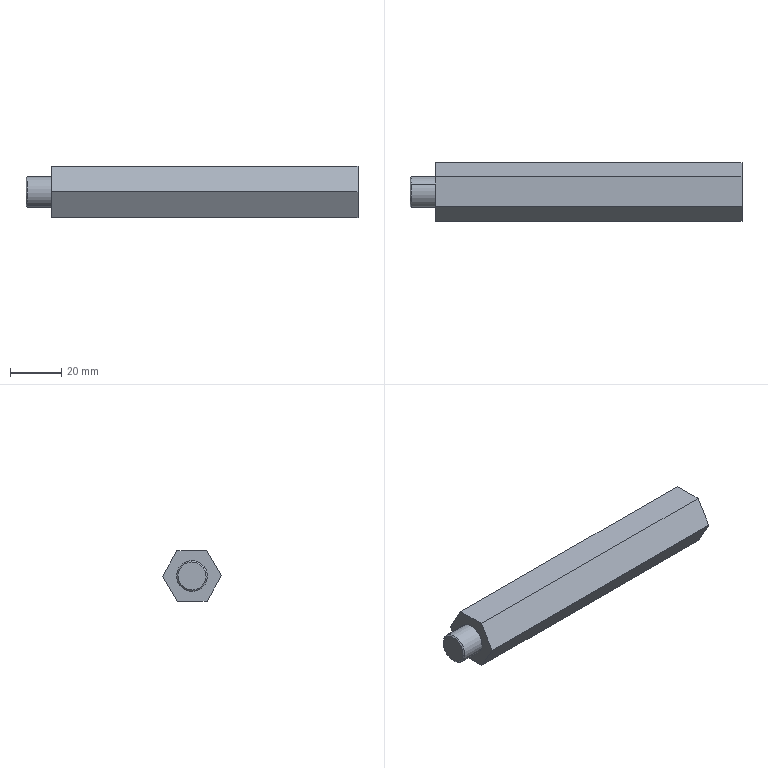Component | SolidWorks | LowerSideBeltXG-XG1-1_RollerMountingPlateABConnectingRodXG-XG1-1 | 1 solid | 17 faces | box 130 x 23.09 x 20.14 mm | volume 41863 mm3 | plane 9 | cone 4 | cylinder 4 | commonest cylinder face diameters 12 x2 6.8 x2
STEP:
#1=COLOUR_RGB('',0.7922,0.8196,0.9333);
#2=FILL_AREA_STYLE_COLOUR('',#1);
#3=FILL_AREA_STYLE('',(#2));
#4=SURFACE_STYLE_FILL_AREA(#3);
#5=SURFACE_SIDE_STYLE('',(#4));
#6=SURFACE_STYLE_USAGE(.BOTH.,#5);
#7=PRESENTATION_STYLE_ASSIGNMENT((#6));
#8=CARTESIAN_POINT('',(-12.843,21.445,3.515));
#9=VERTEX_POINT('',#8);
#10=CARTESIAN_POINT('',(-12.843,21.666,3.887));
#11=VERTEX_POINT('',#10);
#12=CARTESIAN_POINT('',(-12.843,21.555,3.701));
#13=DIRECTION('',(-1.,-0.,0.));
#14=DIRECTION('',(0.,-0.5106,-0.8598));
#15=AXIS2_PLACEMENT_3D('',#12,#13,#14);
#16=CIRCLE('',#15,0.2165);
#17=EDGE_CURVE('',#9,#11,#16,.T.);
#18=ORIENTED_EDGE('',*,*,#17,.F.);
#19=CARTESIAN_POINT('',(-12.824,21.434,3.498));
#20=VERTEX_POINT('',#19);
#21=CARTESIAN_POINT('',(-12.843,21.445,3.515));
#22=DIRECTION('',(0.7071,-0.3611,-0.608));
#23=VECTOR('',#22,39.37);
#24=LINE('',#21,#23);
#25=EDGE_CURVE('',#9,#20,#24,.T.);
#26=ORIENTED_EDGE('',*,*,#25,.T.);
#27=CARTESIAN_POINT('',(-12.824,21.676,3.904));
#28=VERTEX_POINT('',#27);
#29=CARTESIAN_POINT('',(-12.824,21.555,3.701));
#30=DIRECTION('',(1.,0.,-0.));
#31=DIRECTION('',(0.,-0.5106,-0.8598));
#32=AXIS2_PLACEMENT_3D('',#29,#30,#31);
#33=CIRCLE('',#32,0.2362);
#34=EDGE_CURVE('',#28,#20,#33,.T.);
#35=ORIENTED_EDGE('',*,*,#34,.F.);
#36=CARTESIAN_POINT('',(-12.843,21.666,3.887));
#37=DIRECTION('',(0.7071,0.3611,0.608));
#38=VECTOR('',#37,39.37);
#39=LINE('',#36,#38);
#40=EDGE_CURVE('',#11,#28,#39,.T.);
#41=ORIENTED_EDGE('',*,*,#40,.F.);
#42=EDGE_LOOP('',(#18,#26,#35,#41));
#43=FACE_OUTER_BOUND('',#42,.T.);
#44=CARTESIAN_POINT('',(-12.843,21.555,3.701));
#45=DIRECTION('',(1.,0.,-0.));
#46=DIRECTION('',(0.,0.5106,0.8598));
#47=AXIS2_PLACEMENT_3D('',#44,#45,#46);
#48=CONICAL_SURFACE('',#47,0.2165,0.7854);
#49=ADVANCED_FACE('',(#43),#48,.T.);
#50=ORIENTED_EDGE('',*,*,#34,.T.);
#51=CARTESIAN_POINT('',(-12.45,21.434,3.498));
#52=VERTEX_POINT('',#51);
#53=CARTESIAN_POINT('',(-12.843,21.434,3.498));
#54=DIRECTION('',(1.,0.,-0.));
#55=VECTOR('',#54,39.37);
#56=LINE('',#53,#55);
#57=EDGE_CURVE('',#20,#52,#56,.T.);
#58=ORIENTED_EDGE('',*,*,#57,.T.);
#59=CARTESIAN_POINT('',(-12.45,21.676,3.904));
#60=VERTEX_POINT('',#59);
#61=CARTESIAN_POINT('',(-12.45,21.555,3.701));
#62=DIRECTION('',(-1.,-0.,0.));
#63=DIRECTION('',(0.,-0.5106,-0.8598));
#64=AXIS2_PLACEMENT_3D('',#61,#62,#63);
#65=CIRCLE('',#64,0.2362);
#66=EDGE_CURVE('',#52,#60,#65,.T.);
#67=ORIENTED_EDGE('',*,*,#66,.T.);
#68=CARTESIAN_POINT('',(-12.843,21.676,3.904));
#69=DIRECTION('',(1.,0.,-0.));
#70=VECTOR('',#69,39.37);
#71=LINE('',#68,#70);
#72=EDGE_CURVE('',#28,#60,#71,.T.);
#73=ORIENTED_EDGE('',*,*,#72,.F.);
#74=EDGE_LOOP('',(#50,#58,#67,#73));
#75=FACE_OUTER_BOUND('',#74,.T.);
#76=CARTESIAN_POINT('',(-12.843,21.555,3.701));
#77=DIRECTION('',(1.,0.,-0.));
#78=DIRECTION('',(0.,0.5106,0.8598));
#79=AXIS2_PLACEMENT_3D('',#76,#77,#78);
#80=CYLINDRICAL_SURFACE('',#79,0.2362);
#81=ADVANCED_FACE('',(#75),#80,.T.);
#82=CARTESIAN_POINT('',(-8.601,21.487,3.586));
#83=VERTEX_POINT('',#82);
#84=CARTESIAN_POINT('',(-8.601,21.623,3.816));
#85=VERTEX_POINT('',#84);
#86=CARTESIAN_POINT('',(-8.601,21.555,3.701));
#87=DIRECTION('',(1.,0.,-0.));
#88=DIRECTION('',(0.,0.5106,0.8598));
#89=AXIS2_PLACEMENT_3D('',#86,#87,#88);
#90=CIRCLE('',#89,0.1339);
#91=EDGE_CURVE('',#83,#85,#90,.T.);
#92=ORIENTED_EDGE('',*,*,#91,.F.);
#93=CARTESIAN_POINT('',(-7.725,21.487,3.586));
#94=VERTEX_POINT('',#93);
#95=CARTESIAN_POINT('',(-7.725,21.487,3.586));
#96=DIRECTION('',(1.,0.,-0.));
#97=VECTOR('',#96,39.37);
#98=LINE('',#95,#97);
#99=EDGE_CURVE('',#83,#94,#98,.T.);
#100=ORIENTED_EDGE('',*,*,#99,.T.);
#101=CARTESIAN_POINT('',(-7.725,21.623,3.816));
#102=VERTEX_POINT('',#101);
#103=CARTESIAN_POINT('',(-7.725,21.555,3.701));
#104=DIRECTION('',(1.,0.,-0.));
#105=DIRECTION('',(0.,0.5106,0.8598));
#106=AXIS2_PLACEMENT_3D('',#103,#104,#105);
#107=CIRCLE('',#106,0.1339);
#108=EDGE_CURVE('',#94,#102,#107,.T.);
#109=ORIENTED_EDGE('',*,*,#108,.T.);
#110=CARTESIAN_POINT('',(-7.725,21.623,3.816));
#111=DIRECTION('',(1.,0.,-0.));
#112=VECTOR('',#111,39.37);
#113=LINE('',#110,#112);
#114=EDGE_CURVE('',#85,#102,#113,.T.);
#115=ORIENTED_EDGE('',*,*,#114,.F.);
#116=EDGE_LOOP('',(#92,#100,#109,#115));
#117=FACE_OUTER_BOUND('',#116,.T.);
#118=CARTESIAN_POINT('',(-7.725,21.555,3.701));
#119=DIRECTION('',(1.,0.,-0.));
#120=DIRECTION('',(0.,0.5106,0.8598));
#121=AXIS2_PLACEMENT_3D('',#118,#119,#120);
#122=CYLINDRICAL_SURFACE('',#121,0.1339);
#123=ADVANCED_FACE('',(#117),#122,.F.);
#124=CARTESIAN_POINT('',(-8.682,21.555,3.701));
#125=VERTEX_POINT('',#124);
#126=CARTESIAN_POINT('',(-8.601,21.623,3.816));
#127=DIRECTION('',(0.515,0.4377,0.737));
#128=VECTOR('',#127,39.37);
#129=LINE('',#126,#128);
#130=EDGE_CURVE('',#125,#85,#129,.T.);
#131=ORIENTED_EDGE('',*,*,#130,.F.);
#132=CARTESIAN_POINT('',(-8.601,21.487,3.586));
#133=DIRECTION('',(0.515,-0.4377,-0.737));
#134=VECTOR('',#133,39.37);
#135=LINE('',#132,#134);
#136=EDGE_CURVE('',#125,#83,#135,.T.);
#137=ORIENTED_EDGE('',*,*,#136,.T.);
#138=ORIENTED_EDGE('',*,*,#91,.T.);
#139=EDGE_LOOP('',(#131,#137,#138));
#140=FACE_OUTER_BOUND('',#139,.T.);
#141=CARTESIAN_POINT('',(-8.601,21.555,3.701));
#142=DIRECTION('',(1.,0.,-0.));
#143=DIRECTION('',(0.,0.5106,0.8598));
#144=AXIS2_PLACEMENT_3D('',#141,#142,#143);
#145=CONICAL_SURFACE('',#144,0.1339,1.03);
#146=ADVANCED_FACE('',(#140),#145,.F.);
#147=CARTESIAN_POINT('',(-12.45,21.778,3.304));
#148=VERTEX_POINT('',#147);
#149=CARTESIAN_POINT('',(-12.45,21.323,3.31));
#150=VERTEX_POINT('',#149);
#151=CARTESIAN_POINT('',(-12.45,21.778,3.304));
#152=DIRECTION('',(0.,-0.9999,0.01233));
#153=VECTOR('',#152,39.37);
#154=LINE('',#151,#153);
#155=EDGE_CURVE('',#148,#150,#154,.T.);
#156=ORIENTED_EDGE('',*,*,#155,.T.);
#157=CARTESIAN_POINT('',(-12.45,21.101,3.706));
#158=VERTEX_POINT('',#157);
#159=CARTESIAN_POINT('',(-12.45,21.323,3.31));
#160=DIRECTION('',(0.,-0.4893,0.8721));
#161=VECTOR('',#160,39.37);
#162=LINE('',#159,#161);
#163=EDGE_CURVE('',#150,#158,#162,.T.);
#164=ORIENTED_EDGE('',*,*,#163,.T.);
#165=CARTESIAN_POINT('',(-12.45,21.333,4.097));
#166=VERTEX_POINT('',#165);
#167=CARTESIAN_POINT('',(-12.45,21.101,3.706));
#168=DIRECTION('',(-0.,0.5106,0.8598));
#169=VECTOR('',#168,39.37);
#170=LINE('',#167,#169);
#171=EDGE_CURVE('',#158,#166,#170,.T.);
#172=ORIENTED_EDGE('',*,*,#171,.T.);
#173=CARTESIAN_POINT('',(-12.45,21.787,4.092));
#174=VERTEX_POINT('',#173);
#175=CARTESIAN_POINT('',(-12.45,21.333,4.097));
#176=DIRECTION('',(-0.,0.9999,-0.01233));
#177=VECTOR('',#176,39.37);
#178=LINE('',#175,#177);
#179=EDGE_CURVE('',#166,#174,#178,.T.);
#180=ORIENTED_EDGE('',*,*,#179,.T.);
#181=CARTESIAN_POINT('',(-12.45,22.01,3.695));
#182=VERTEX_POINT('',#181);
#183=CARTESIAN_POINT('',(-12.45,21.787,4.092));
#184=DIRECTION('',(-0.,0.4893,-0.8721));
#185=VECTOR('',#184,39.37);
#186=LINE('',#183,#185);
#187=EDGE_CURVE('',#174,#182,#186,.T.);
#188=ORIENTED_EDGE('',*,*,#187,.T.);
#189=CARTESIAN_POINT('',(-12.45,22.01,3.695));
#190=DIRECTION('',(0.,-0.5106,-0.8598));
#191=VECTOR('',#190,39.37);
#192=LINE('',#189,#191);
#193=EDGE_CURVE('',#182,#148,#192,.T.);
#194=ORIENTED_EDGE('',*,*,#193,.T.);
#195=EDGE_LOOP('',(#156,#164,#172,#180,#188,#194));
#196=FACE_OUTER_BOUND('',#195,.T.);
#197=CARTESIAN_POINT('',(-12.45,21.555,3.701));
#198=DIRECTION('',(-1.,-0.,0.));
#199=DIRECTION('',(0.,-0.5106,-0.8598));
#200=AXIS2_PLACEMENT_3D('',#197,#198,#199);
#201=CIRCLE('',#200,0.2362);
#202=EDGE_CURVE('',#60,#52,#201,.T.);
#203=ORIENTED_EDGE('',*,*,#202,.F.);
#204=ORIENTED_EDGE('',*,*,#66,.F.);
#205=EDGE_LOOP('',(#203,#204));
#206=FACE_BOUND('',#205,.T.);
#207=CARTESIAN_POINT('',(-12.45,21.555,3.701));
#208=DIRECTION('',(-1.,-0.,0.));
#209=DIRECTION('',(0.,-0.5106,-0.8598));
#210=AXIS2_PLACEMENT_3D('',#207,#208,#209);
#211=PLANE('',#210);
#212=ADVANCED_FACE('',(#196,#206),#211,.T.);
#213=CARTESIAN_POINT('',(-7.725,21.778,3.304));
#214=VERTEX_POINT('',#213);
#215=CARTESIAN_POINT('',(-7.725,21.323,3.31));
#216=VERTEX_POINT('',#215);
#217=CARTESIAN_POINT('',(-7.725,21.778,3.304));
#218=DIRECTION('',(0.,-0.9999,0.01233));
#219=VECTOR('',#218,39.37);
#220=LINE('',#217,#219);
#221=EDGE_CURVE('',#214,#216,#220,.T.);
#222=ORIENTED_EDGE('',*,*,#221,.T.);
#223=CARTESIAN_POINT('',(-12.45,21.323,3.31));
#224=DIRECTION('',(1.,0.,-0.));
#225=VECTOR('',#224,39.37);
#226=LINE('',#223,#225);
#227=EDGE_CURVE('',#150,#216,#226,.T.);
#228=ORIENTED_EDGE('',*,*,#227,.F.);
#229=ORIENTED_EDGE('',*,*,#155,.F.);
#230=CARTESIAN_POINT('',(-12.45,21.778,3.304));
#231=DIRECTION('',(1.,0.,-0.));
#232=VECTOR('',#231,39.37);
#233=LINE('',#230,#232);
#234=EDGE_CURVE('',#148,#214,#233,.T.);
#235=ORIENTED_EDGE('',*,*,#234,.T.);
#236=EDGE_LOOP('',(#222,#228,#229,#235));
#237=FACE_OUTER_BOUND('',#236,.T.);
#238=CARTESIAN_POINT('',(-12.45,21.778,3.304));
#239=DIRECTION('',(-0.,0.01233,0.9999));
#240=DIRECTION('',(-0.,0.9999,-0.01233));
#241=AXIS2_PLACEMENT_3D('',#238,#239,#240);
#242=PLANE('',#241);
#243=ADVANCED_FACE('',(#237),#242,.F.);
#244=CARTESIAN_POINT('',(-7.725,21.101,3.706));
#245=VERTEX_POINT('',#244);
#246=CARTESIAN_POINT('',(-7.725,21.323,3.31));
#247=DIRECTION('',(0.,-0.4893,0.8721));
#248=VECTOR('',#247,39.37);
#249=LINE('',#246,#248);
#250=EDGE_CURVE('',#216,#245,#249,.T.);
#251=ORIENTED_EDGE('',*,*,#250,.T.);
#252=CARTESIAN_POINT('',(-12.45,21.101,3.706));
#253=DIRECTION('',(1.,0.,-0.));
#254=VECTOR('',#253,39.37);
#255=LINE('',#252,#254);
#256=EDGE_CURVE('',#158,#245,#255,.T.);
#257=ORIENTED_EDGE('',*,*,#256,.F.);
#258=ORIENTED_EDGE('',*,*,#163,.F.);
#259=ORIENTED_EDGE('',*,*,#227,.T.);
#260=EDGE_LOOP('',(#251,#257,#258,#259));
#261=FACE_OUTER_BOUND('',#260,.T.);
#262=CARTESIAN_POINT('',(-12.45,21.323,3.31));
#263=DIRECTION('',(-0.,0.8721,0.4893));
#264=DIRECTION('',(-0.,0.4893,-0.8721));
#265=AXIS2_PLACEMENT_3D('',#262,#263,#264);
#266=PLANE('',#265);
#267=ADVANCED_FACE('',(#261),#266,.F.);
#268=CARTESIAN_POINT('',(-7.725,21.333,4.097));
#269=VERTEX_POINT('',#268);
#270=CARTESIAN_POINT('',(-7.725,21.101,3.706));
#271=DIRECTION('',(-0.,0.5106,0.8598));
#272=VECTOR('',#271,39.37);
#273=LINE('',#270,#272);
#274=EDGE_CURVE('',#245,#269,#273,.T.);
#275=ORIENTED_EDGE('',*,*,#274,.T.);
#276=CARTESIAN_POINT('',(-12.45,21.333,4.097));
#277=DIRECTION('',(1.,0.,-0.));
#278=VECTOR('',#277,39.37);
#279=LINE('',#276,#278);
#280=EDGE_CURVE('',#166,#269,#279,.T.);
#281=ORIENTED_EDGE('',*,*,#280,.F.);
#282=ORIENTED_EDGE('',*,*,#171,.F.);
#283=ORIENTED_EDGE('',*,*,#256,.T.);
#284=EDGE_LOOP('',(#275,#281,#282,#283));
#285=FACE_OUTER_BOUND('',#284,.T.);
#286=CARTESIAN_POINT('',(-12.45,21.101,3.706));
#287=DIRECTION('',(-0.,0.8598,-0.5106));
#288=DIRECTION('',(0.,-0.5106,-0.8598));
#289=AXIS2_PLACEMENT_3D('',#286,#287,#288);
#290=PLANE('',#289);
#291=ADVANCED_FACE('',(#285),#290,.F.);
#292=CARTESIAN_POINT('',(-7.725,21.787,4.092));
#293=VERTEX_POINT('',#292);
#294=CARTESIAN_POINT('',(-7.725,21.333,4.097));
#295=DIRECTION('',(-0.,0.9999,-0.01233));
#296=VECTOR('',#295,39.37);
#297=LINE('',#294,#296);
#298=EDGE_CURVE('',#269,#293,#297,.T.);
#299=ORIENTED_EDGE('',*,*,#298,.T.);
#300=CARTESIAN_POINT('',(-12.45,21.787,4.092));
#301=DIRECTION('',(1.,0.,-0.));
#302=VECTOR('',#301,39.37);
#303=LINE('',#300,#302);
#304=EDGE_CURVE('',#174,#293,#303,.T.);
#305=ORIENTED_EDGE('',*,*,#304,.F.);
#306=ORIENTED_EDGE('',*,*,#179,.F.);
#307=ORIENTED_EDGE('',*,*,#280,.T.);
#308=EDGE_LOOP('',(#299,#305,#306,#307));
#309=FACE_OUTER_BOUND('',#308,.T.);
#310=CARTESIAN_POINT('',(-12.45,21.333,4.097));
#311=DIRECTION('',(0.,-0.01233,-0.9999));
#312=DIRECTION('',(0.,-0.9999,0.01233));
#313=AXIS2_PLACEMENT_3D('',#310,#311,#312);
#314=PLANE('',#313);
#315=ADVANCED_FACE('',(#309),#314,.F.);
#316=CARTESIAN_POINT('',(-7.725,22.01,3.695));
#317=VERTEX_POINT('',#316);
#318=CARTESIAN_POINT('',(-7.725,21.787,4.092));
#319=DIRECTION('',(-0.,0.4893,-0.8721));
#320=VECTOR('',#319,39.37);
#321=LINE('',#318,#320);
#322=EDGE_CURVE('',#293,#317,#321,.T.);
#323=ORIENTED_EDGE('',*,*,#322,.T.);
#324=CARTESIAN_POINT('',(-12.45,22.01,3.695));
#325=DIRECTION('',(1.,0.,-0.));
#326=VECTOR('',#325,39.37);
#327=LINE('',#324,#326);
#328=EDGE_CURVE('',#182,#317,#327,.T.);
#329=ORIENTED_EDGE('',*,*,#328,.F.);
#330=ORIENTED_EDGE('',*,*,#187,.F.);
#331=ORIENTED_EDGE('',*,*,#304,.T.);
#332=EDGE_LOOP('',(#323,#329,#330,#331));
#333=FACE_OUTER_BOUND('',#332,.T.);
#334=CARTESIAN_POINT('',(-12.45,21.787,4.092));
#335=DIRECTION('',(0.,-0.8721,-0.4893));
#336=DIRECTION('',(0.,-0.4893,0.8721));
#337=AXIS2_PLACEMENT_3D('',#334,#335,#336);
#338=PLANE('',#337);
#339=ADVANCED_FACE('',(#333),#338,.F.);
#340=CARTESIAN_POINT('',(-7.725,22.01,3.695));
#341=DIRECTION('',(0.,-0.5106,-0.8598));
#342=VECTOR('',#341,39.37);
#343=LINE('',#340,#342);
#344=EDGE_CURVE('',#317,#214,#343,.T.);
#345=ORIENTED_EDGE('',*,*,#344,.T.);
#346=ORIENTED_EDGE('',*,*,#234,.F.);
#347=ORIENTED_EDGE('',*,*,#193,.F.);
#348=ORIENTED_EDGE('',*,*,#328,.T.);
#349=EDGE_LOOP('',(#345,#346,#347,#348));
#350=FACE_OUTER_BOUND('',#349,.T.);
#351=CARTESIAN_POINT('',(-12.45,22.01,3.695));
#352=DIRECTION('',(0.,-0.8598,0.5106));
#353=DIRECTION('',(-0.,0.5106,0.8598));
#354=AXIS2_PLACEMENT_3D('',#351,#352,#353);
#355=PLANE('',#354);
#356=ADVANCED_FACE('',(#350),#355,.F.);
#357=CARTESIAN_POINT('',(-7.725,21.555,3.701));
#358=DIRECTION('',(1.,0.,-0.));
#359=DIRECTION('',(0.,0.5106,0.8598));
#360=AXIS2_PLACEMENT_3D('',#357,#358,#359);
#361=CIRCLE('',#360,0.1339);
#362=EDGE_CURVE('',#102,#94,#361,.T.);
#363=ORIENTED_EDGE('',*,*,#362,.F.);
#364=ORIENTED_EDGE('',*,*,#108,.F.);
#365=EDGE_LOOP('',(#363,#364));
#366=FACE_BOUND('',#365,.T.);
#367=ORIENTED_EDGE('',*,*,#221,.F.);
#368=ORIENTED_EDGE('',*,*,#344,.F.);
#369=ORIENTED_EDGE('',*,*,#322,.F.);
#370=ORIENTED_EDGE('',*,*,#298,.F.);
#371=ORIENTED_EDGE('',*,*,#274,.F.);
#372=ORIENTED_EDGE('',*,*,#250,.F.);
#373=EDGE_LOOP('',(#367,#368,#369,#370,#371,#372));
#374=FACE_OUTER_BOUND('',#373,.T.);
#375=CARTESIAN_POINT('',(-7.725,21.555,3.701));
#376=DIRECTION('',(-1.,-0.,0.));
#377=DIRECTION('',(0.,-0.5106,-0.8598));
#378=AXIS2_PLACEMENT_3D('',#375,#376,#377);
#379=PLANE('',#378);
#380=ADVANCED_FACE('',(#366,#374),#379,.F.);
#381=ORIENTED_EDGE('',*,*,#136,.F.);
#382=ORIENTED_EDGE('',*,*,#130,.T.);
#383=CARTESIAN_POINT('',(-8.601,21.555,3.701));
#384=DIRECTION('',(1.,0.,-0.));
#385=DIRECTION('',(0.,0.5106,0.8598));
#386=AXIS2_PLACEMENT_3D('',#383,#384,#385);
#387=CIRCLE('',#386,0.1339);
#388=EDGE_CURVE('',#85,#83,#387,.T.);
#389=ORIENTED_EDGE('',*,*,#388,.T.);
#390=EDGE_LOOP('',(#381,#382,#389));
#391=FACE_OUTER_BOUND('',#390,.T.);
#392=CARTESIAN_POINT('',(-8.601,21.555,3.701));
#393=DIRECTION('',(1.,0.,-0.));
#394=DIRECTION('',(0.,0.5106,0.8598));
#395=AXIS2_PLACEMENT_3D('',#392,#393,#394);
#396=CONICAL_SURFACE('',#395,0.1339,1.03);
#397=ADVANCED_FACE('',(#391),#396,.F.);
#398=ORIENTED_EDGE('',*,*,#99,.F.);
#399=ORIENTED_EDGE('',*,*,#388,.F.);
#400=ORIENTED_EDGE('',*,*,#114,.T.);
#401=ORIENTED_EDGE('',*,*,#362,.T.);
#402=EDGE_LOOP('',(#398,#399,#400,#401));
#403=FACE_OUTER_BOUND('',#402,.T.);
#404=CARTESIAN_POINT('',(-7.725,21.555,3.701));
#405=DIRECTION('',(1.,0.,-0.));
#406=DIRECTION('',(0.,0.5106,0.8598));
#407=AXIS2_PLACEMENT_3D('',#404,#405,#406);
#408=CYLINDRICAL_SURFACE('',#407,0.1339);
#409=ADVANCED_FACE('',(#403),#408,.F.);
#410=ORIENTED_EDGE('',*,*,#57,.F.);
#411=CARTESIAN_POINT('',(-12.824,21.555,3.701));
#412=DIRECTION('',(1.,0.,-0.));
#413=DIRECTION('',(0.,-0.5106,-0.8598));
#414=AXIS2_PLACEMENT_3D('',#411,#412,#413);
#415=CIRCLE('',#414,0.2362);
#416=EDGE_CURVE('',#20,#28,#415,.T.);
#417=ORIENTED_EDGE('',*,*,#416,.T.);
#418=ORIENTED_EDGE('',*,*,#72,.T.);
#419=ORIENTED_EDGE('',*,*,#202,.T.);
#420=EDGE_LOOP('',(#410,#417,#418,#419));
#421=FACE_OUTER_BOUND('',#420,.T.);
#422=CARTESIAN_POINT('',(-12.843,21.555,3.701));
#423=DIRECTION('',(1.,0.,-0.));
#424=DIRECTION('',(0.,0.5106,0.8598));
#425=AXIS2_PLACEMENT_3D('',#422,#423,#424);
#426=CYLINDRICAL_SURFACE('',#425,0.2362);
#427=ADVANCED_FACE('',(#421),#426,.T.);
#428=CARTESIAN_POINT('',(-12.843,21.555,3.701));
#429=DIRECTION('',(-1.,-0.,0.));
#430=DIRECTION('',(0.,-0.5106,-0.8598));
#431=AXIS2_PLACEMENT_3D('',#428,#429,#430);
#432=CIRCLE('',#431,0.2165);
#433=EDGE_CURVE('',#11,#9,#432,.T.);
#434=ORIENTED_EDGE('',*,*,#433,.T.);
#435=ORIENTED_EDGE('',*,*,#17,.T.);
#436=EDGE_LOOP('',(#434,#435));
#437=FACE_OUTER_BOUND('',#436,.T.);
#438=CARTESIAN_POINT('',(-12.843,21.555,3.701));
#439=DIRECTION('',(-1.,-0.,0.));
#440=DIRECTION('',(0.,-0.5106,-0.8598));
#441=AXIS2_PLACEMENT_3D('',#438,#439,#440);
#442=PLANE('',#441);
#443=ADVANCED_FACE('',(#437),#442,.T.);
#444=ORIENTED_EDGE('',*,*,#25,.F.);
#445=ORIENTED_EDGE('',*,*,#433,.F.);
#446=ORIENTED_EDGE('',*,*,#40,.T.);
#447=ORIENTED_EDGE('',*,*,#416,.F.);
#448=EDGE_LOOP('',(#444,#445,#446,#447));
#449=FACE_OUTER_BOUND('',#448,.T.);
#450=CARTESIAN_POINT('',(-12.843,21.555,3.701));
#451=DIRECTION('',(1.,0.,-0.));
#452=DIRECTION('',(0.,0.5106,0.8598));
#453=AXIS2_PLACEMENT_3D('',#450,#451,#452);
#454=CONICAL_SURFACE('',#453,0.2165,0.7854);
#455=ADVANCED_FACE('',(#449),#454,.T.);
#456=CLOSED_SHELL('',(#49,#81,#123,#146,#212,#243,#267,#291,#315,#339,#356,#380,#397,#409,#427,#443,#455));
#457=MANIFOLD_SOLID_BREP('',#456);
#458=STYLED_ITEM('',(#7),#457);
#459=PRESENTATION_LAYER_ASSIGNMENT('','',(#458));
#460=CARTESIAN_POINT('',(0.,0.,0.));
#461=DIRECTION('',(0.,0.,1.));
#462=DIRECTION('',(1.,0.,0.));
#463=AXIS2_PLACEMENT_3D('',#460,#461,#462);
#464=(LENGTH_UNIT()NAMED_UNIT(*)SI_UNIT($,.METRE.));
#465=LENGTH_MEASURE_WITH_UNIT(LENGTH_MEASURE(0.0254),#464);
#466=DIMENSIONAL_EXPONENTS(1.,0.,0.,0.,0.,0.,0.);
#467=(CONVERSION_BASED_UNIT('',#465)LENGTH_UNIT()NAMED_UNIT(#466));
#468=UNCERTAINTY_MEASURE_WITH_UNIT(LENGTH_MEASURE(0.00001),#467,'','');
#469=(NAMED_UNIT(*)PLANE_ANGLE_UNIT()SI_UNIT($,.RADIAN.));
#470=(NAMED_UNIT(*)SI_UNIT($,.STERADIAN.)SOLID_ANGLE_UNIT());
#471=(GEOMETRIC_REPRESENTATION_CONTEXT(3)GLOBAL_UNCERTAINTY_ASSIGNED_CONTEXT((#468))GLOBAL_UNIT_ASSIGNED_CONTEXT((#467,#469,#470))REPRESENTATION_CONTEXT('',''));
#472=ADVANCED_BREP_SHAPE_REPRESENTATION('',(#457,#463),#471);
#473=(LENGTH_UNIT()NAMED_UNIT(*)SI_UNIT($,.METRE.));
#474=LENGTH_MEASURE_WITH_UNIT(LENGTH_MEASURE(0.0254),#473);
#475=DIMENSIONAL_EXPONENTS(1.,0.,0.,0.,0.,0.,0.);
#476=(CONVERSION_BASED_UNIT('',#474)LENGTH_UNIT()NAMED_UNIT(#475));
#477=UNCERTAINTY_MEASURE_WITH_UNIT(LENGTH_MEASURE(0.00001),#476,'','');
#478=(NAMED_UNIT(*)PLANE_ANGLE_UNIT()SI_UNIT($,.RADIAN.));
#479=(NAMED_UNIT(*)SI_UNIT($,.STERADIAN.)SOLID_ANGLE_UNIT());
#480=(GEOMETRIC_REPRESENTATION_CONTEXT(3)GLOBAL_UNCERTAINTY_ASSIGNED_CONTEXT((#477))GLOBAL_UNIT_ASSIGNED_CONTEXT((#476,#478,#479))REPRESENTATION_CONTEXT('',''));
#481=MECHANICAL_DESIGN_GEOMETRIC_PRESENTATION_REPRESENTATION('',(#458),#480);